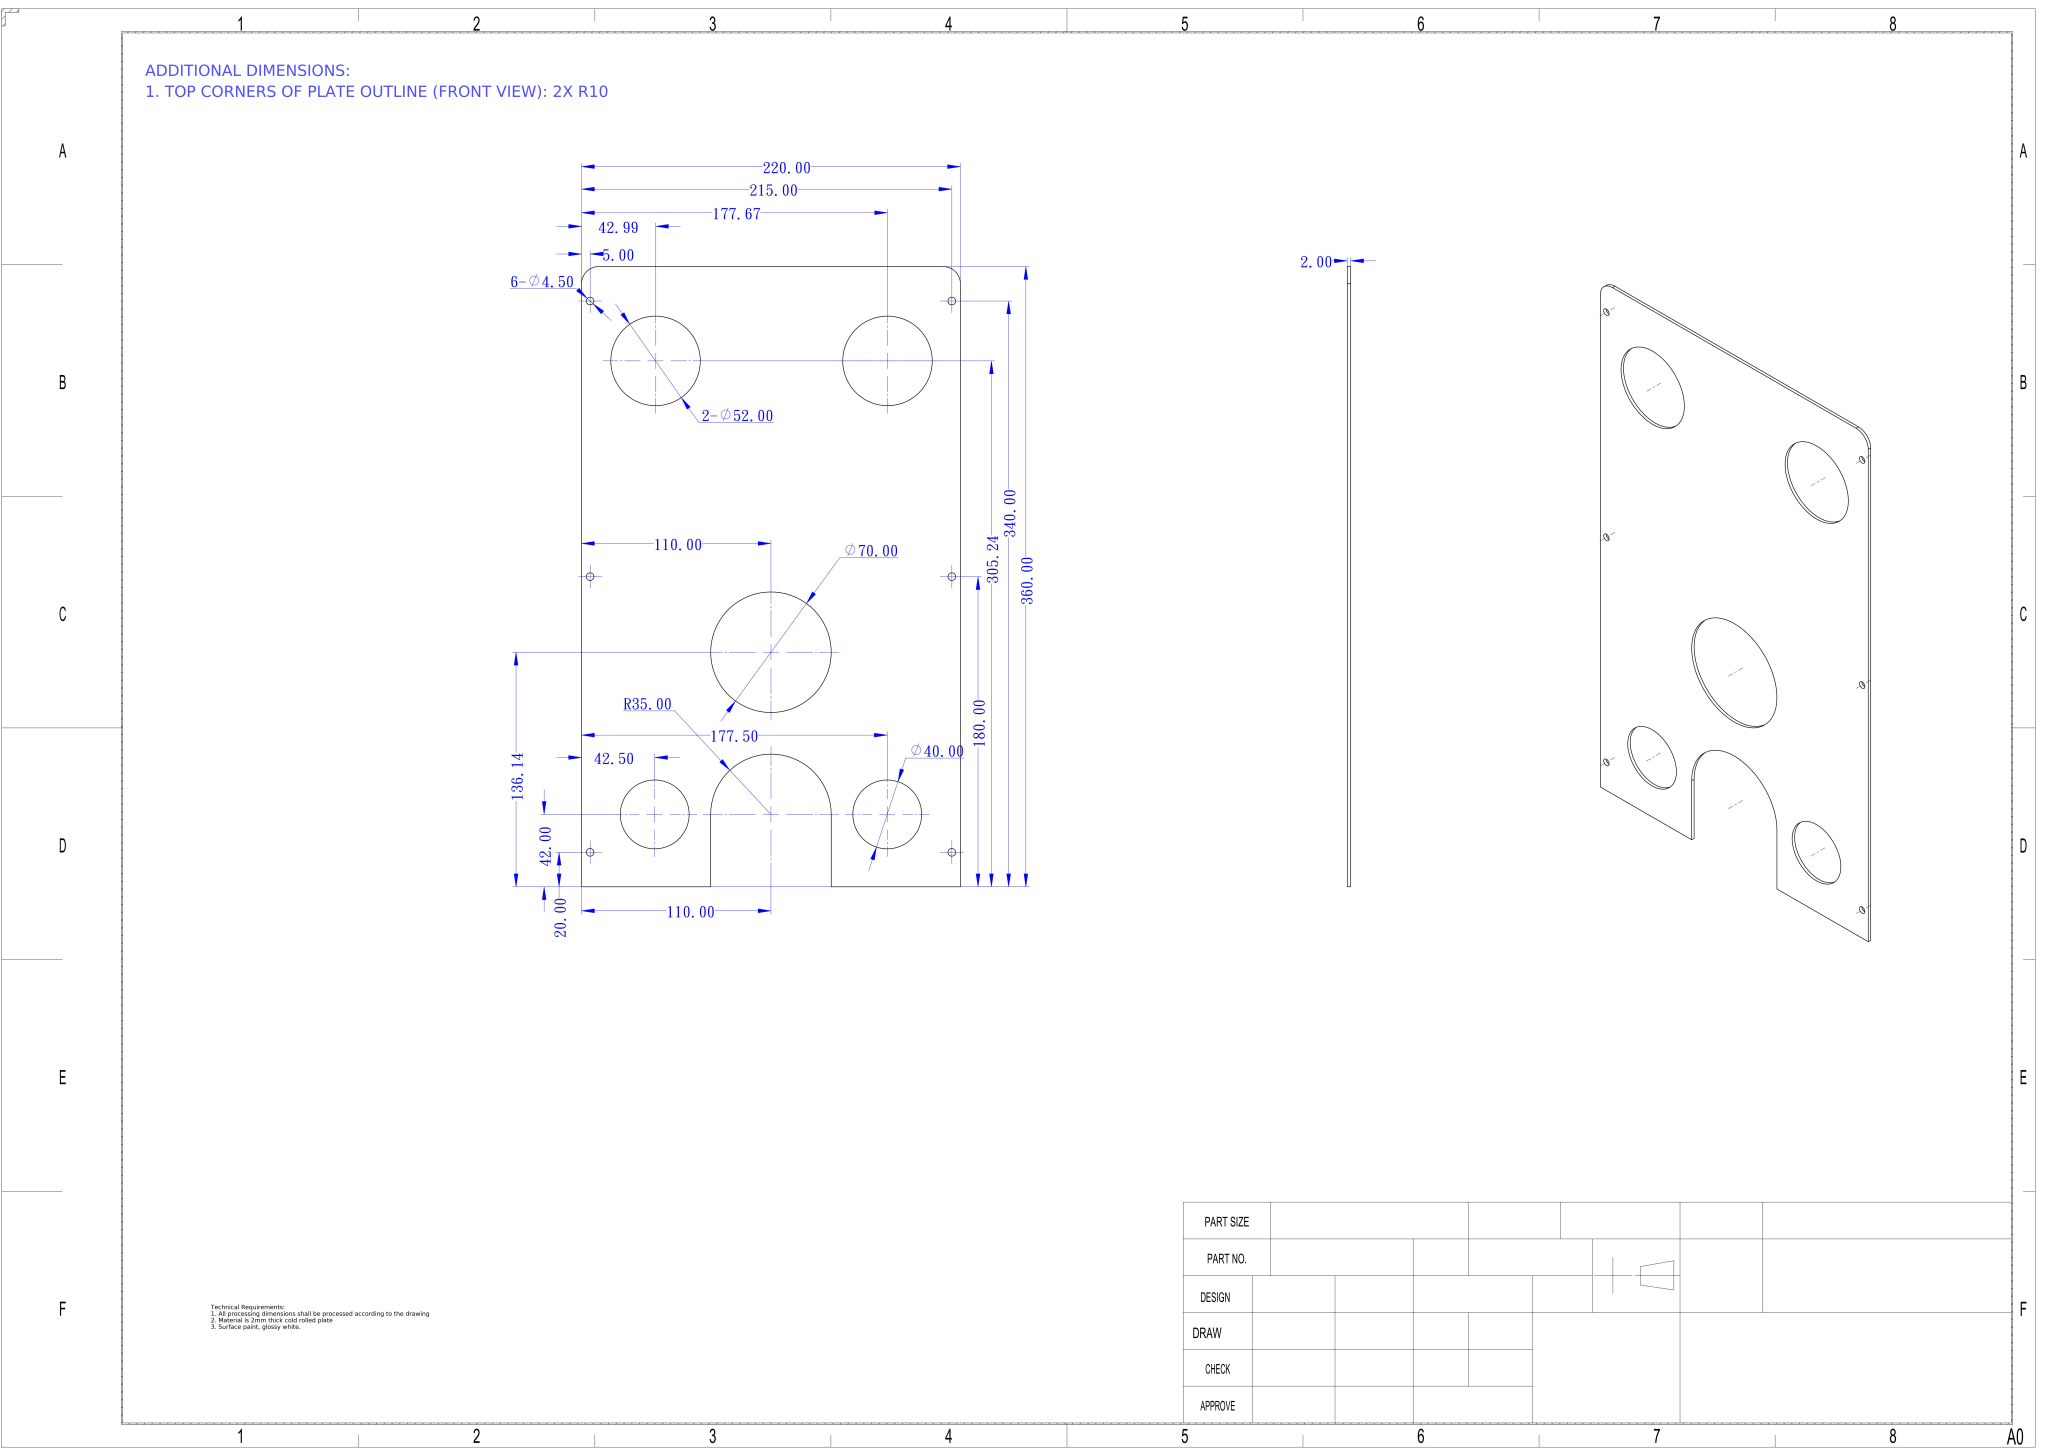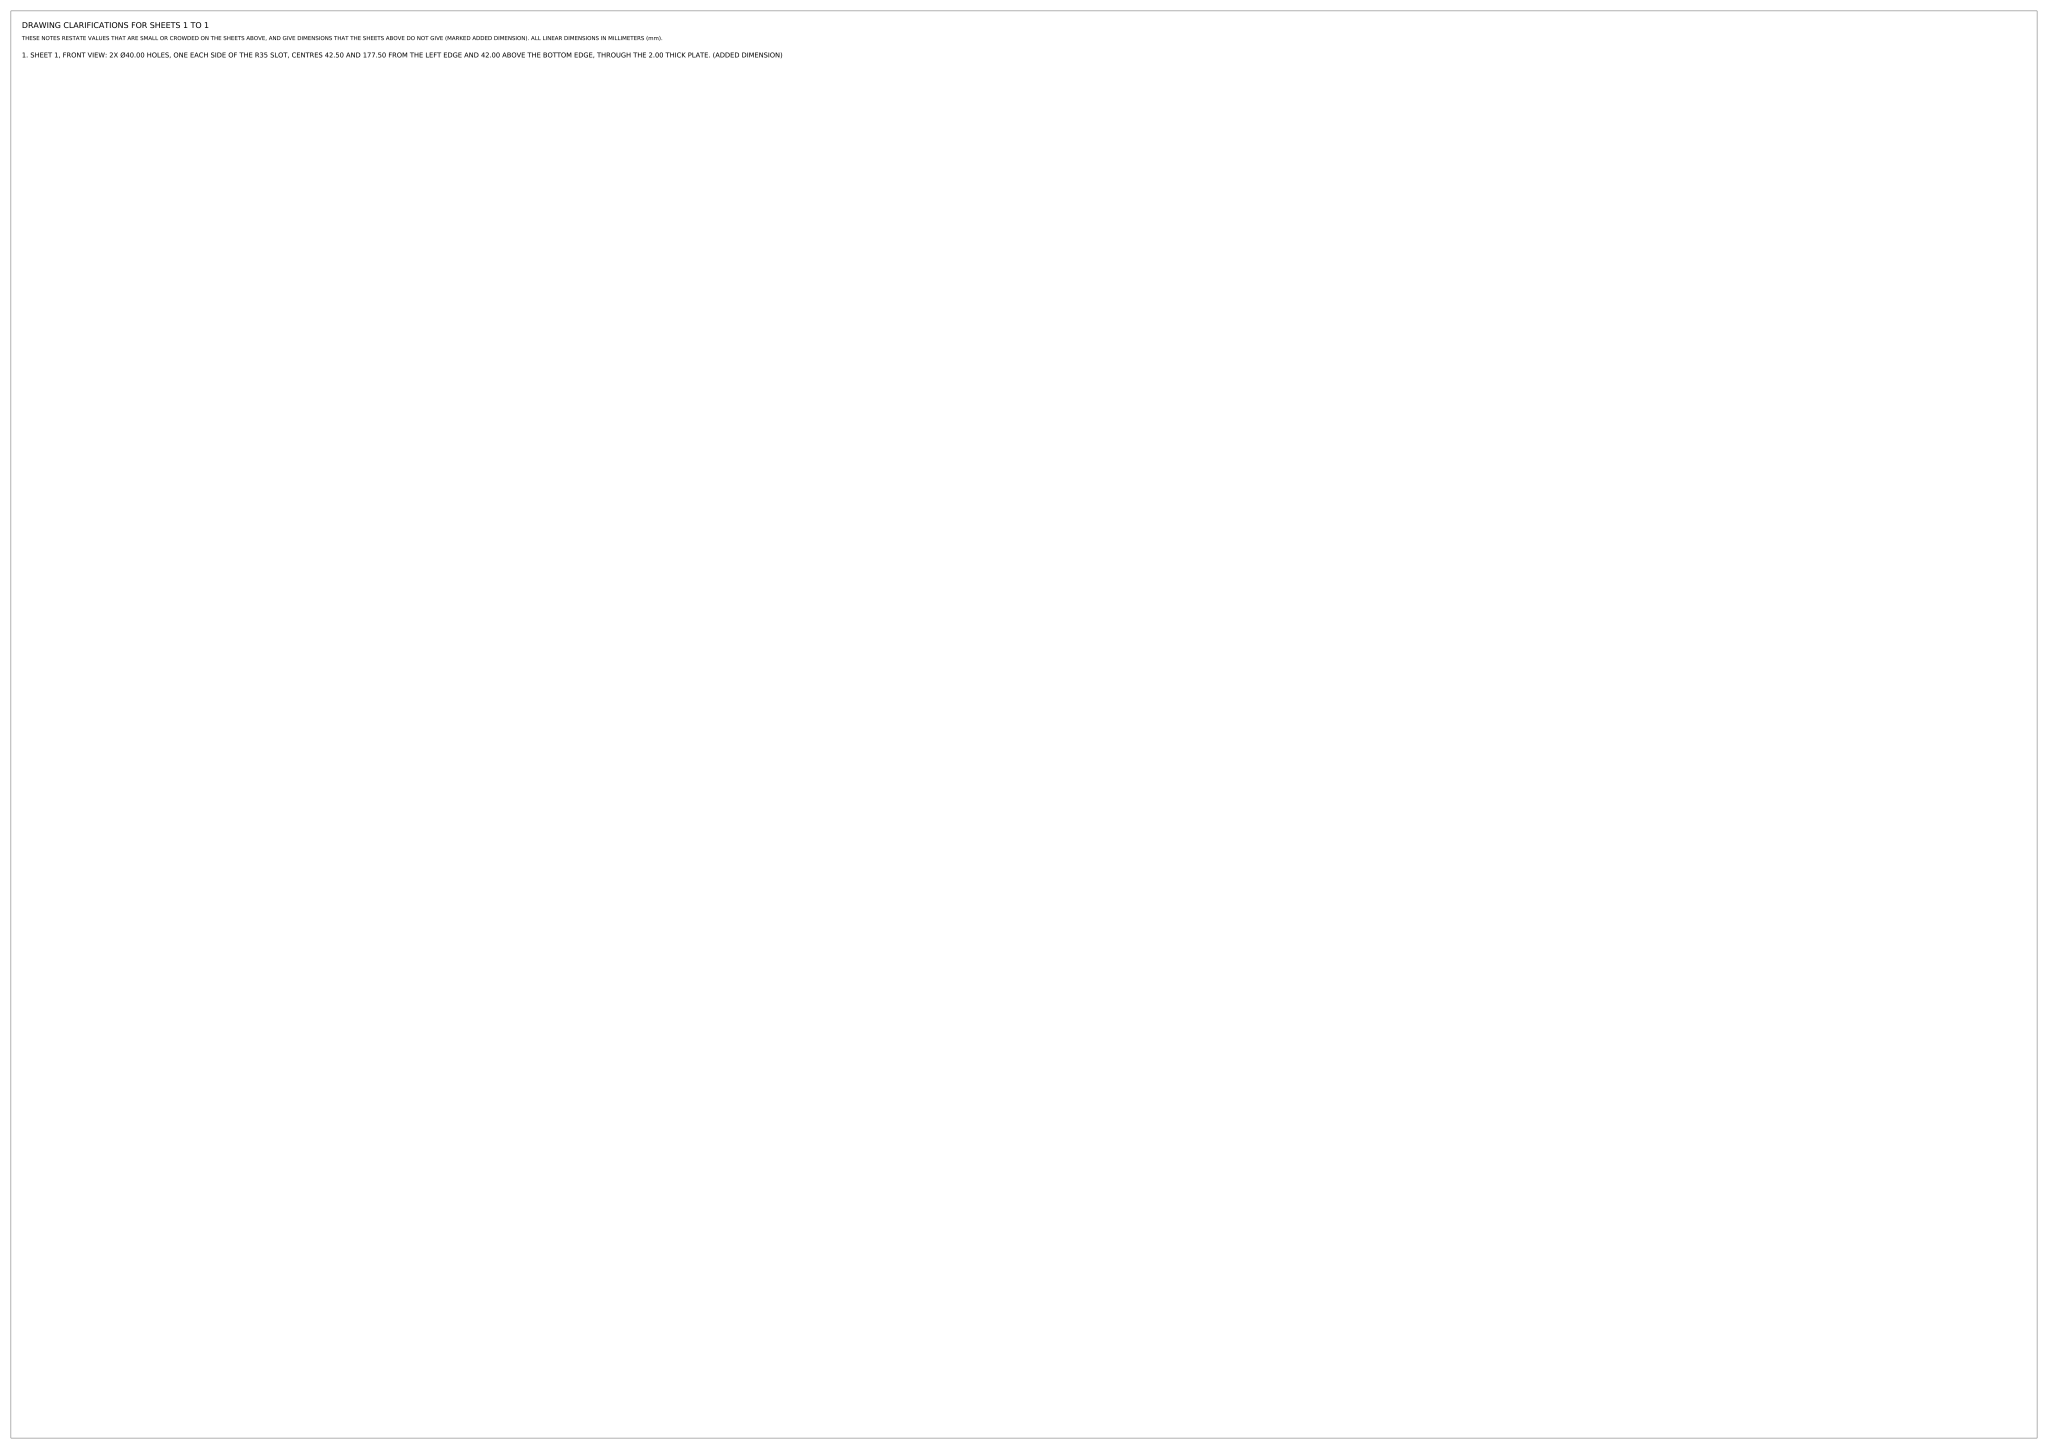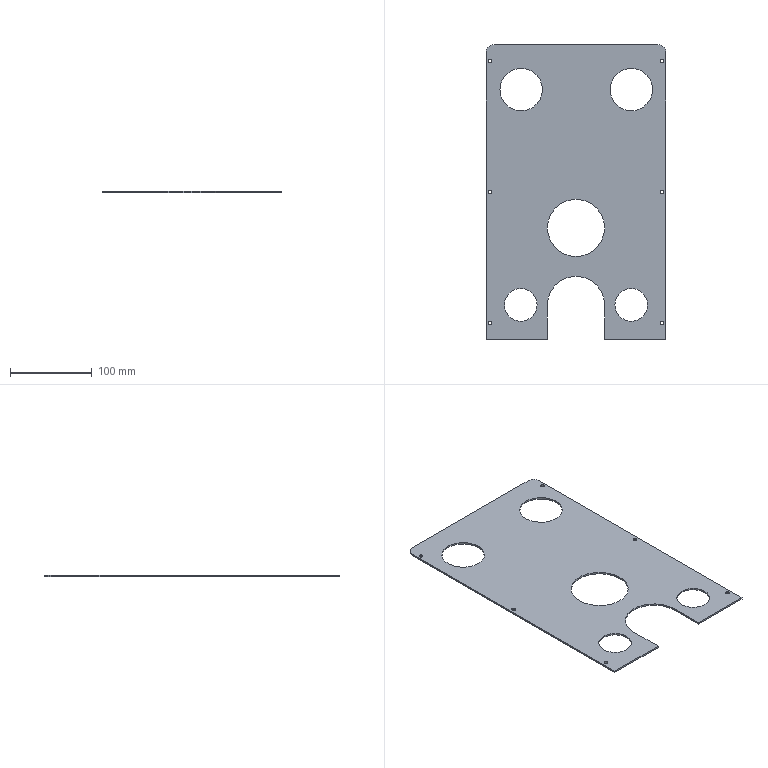Part | NX | mm | 1 solid | 34 faces | box 220 x 360 x 2 mm | volume 127177 mm3 | cylinder 25 | plane 9 | commonest cylinder face diameters 4.5 x12 40 x4 52 x4 70 x3 20 x2